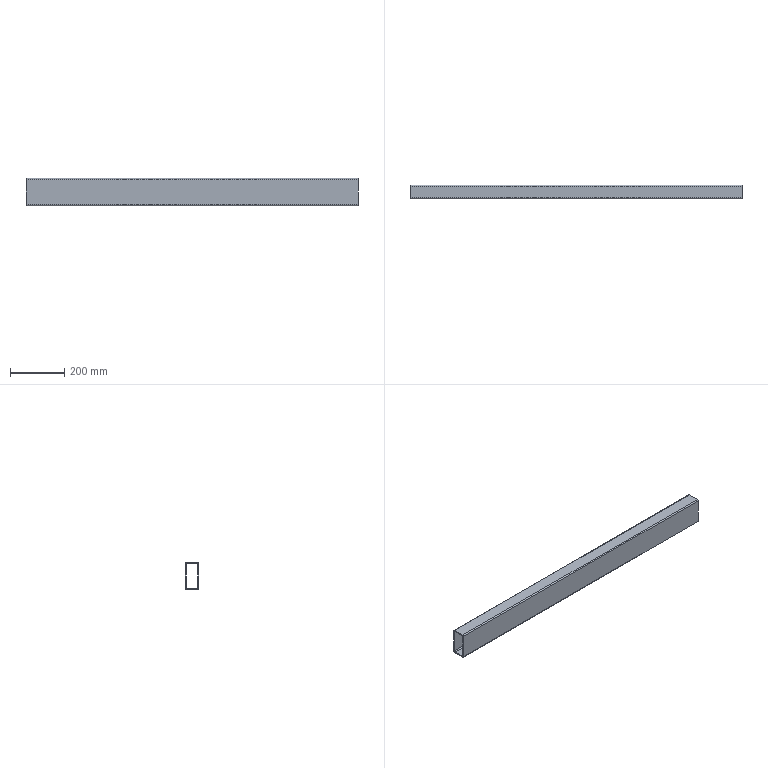Component | NX | BASE_FRAME_RECT_TUBE2 | 1 solid | 18 faces | volume 1391600 mm3 | plane 10 | cylinder 8 | commonest cylinder face diameters 8 x8